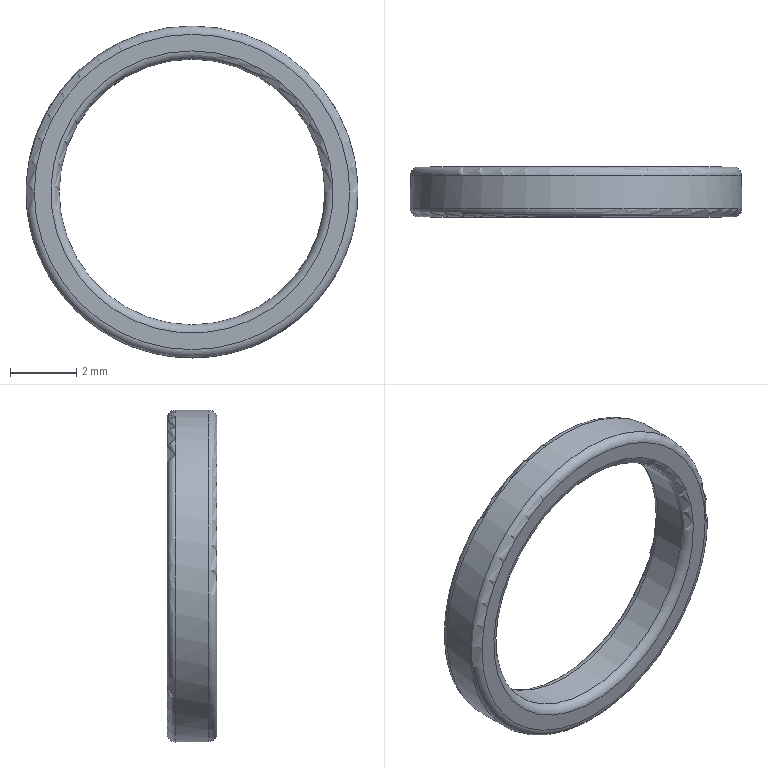Component | NX | AXLESPEEDWASHER | 1 solid | 8 faces | box 10 x 1.5 x 10 mm | volume 41 mm3 | torus 4 | plane 2 | cylinder 2 | commonest cylinder face diameters 10 x1 8 x1
STEP:
#1=CARTESIAN_POINT('',(0.,0.,0.));
#2=DIRECTION('',(0.,0.,1.));
#3=DIRECTION('',(1.,0.,0.));
#4=AXIS2_PLACEMENT_3D('',#1,#2,#3);
#5=CARTESIAN_POINT('',(-422.274,-112.,-59.25));
#6=VERTEX_POINT('',#5);
#7=CARTESIAN_POINT('',(-422.274,-112.,-63.5));
#8=DIRECTION('',(0.,1.,0.));
#9=DIRECTION('',(0.,0.,1.));
#10=AXIS2_PLACEMENT_3D('',#7,#8,#9);
#11=CIRCLE('',#10,4.25);
#12=CARTESIAN_POINT('',(-422.274,-112.,-63.5));
#13=DIRECTION('',(0.,-1.,0.));
#14=DIRECTION('',(0.,0.,1.));
#15=AXIS2_PLACEMENT_3D('',#12,#13,#14);
#16=PLANE('',#15);
#17=CARTESIAN_POINT('',(4.25,0.));
#18=CARTESIAN_POINT('',(4.25,-7.361));
#19=CARTESIAN_POINT('',(-2.125,-3.681));
#20=CARTESIAN_POINT('',(-8.5,-0.));
#21=CARTESIAN_POINT('',(-2.125,3.681));
#22=CARTESIAN_POINT('',(4.25,7.361));
#23=CARTESIAN_POINT('',(4.25,0.));
#24=(BOUNDED_CURVE()B_SPLINE_CURVE(2,(#17,#18,#19,#20,#21,#22,#23),.UNSPECIFIED.,.T.,.F.)B_SPLINE_CURVE_WITH_KNOTS((1,2,2,2,2,1),(-2.094,0.,2.094,4.189,6.283,8.378),.UNSPECIFIED.)CURVE()GEOMETRIC_REPRESENTATION_ITEM()RATIONAL_B_SPLINE_CURVE((1.,0.5,1.,0.5,1.,0.5,1.))REPRESENTATION_ITEM(''));
#25=(GEOMETRIC_REPRESENTATION_CONTEXT(2)PARAMETRIC_REPRESENTATION_CONTEXT()REPRESENTATION_CONTEXT('',''));
#26=DEFINITIONAL_REPRESENTATION('',(#24),#25);
#27=PCURVE('',#16,#26);
#28=CARTESIAN_POINT('',(-422.274,-111.75,-63.5));
#29=DIRECTION('',(0.,-1.,0.));
#30=DIRECTION('',(0.,0.,1.));
#31=AXIS2_PLACEMENT_3D('',#28,#29,#30);
#32=TOROIDAL_SURFACE('',#31,4.25,0.25);
#33=CARTESIAN_POINT('',(6.283,7.854));
#34=DIRECTION('',(-1.,0.));
#35=VECTOR('',#34,1.);
#36=LINE('',#33,#35);
#37=(GEOMETRIC_REPRESENTATION_CONTEXT(2)PARAMETRIC_REPRESENTATION_CONTEXT()REPRESENTATION_CONTEXT('',''));
#38=DEFINITIONAL_REPRESENTATION('',(#36),#37);
#39=PCURVE('',#32,#38);
#40=SURFACE_CURVE('',#11,(#27,#39),.PCURVE_S1.);
#41=EDGE_CURVE('',#6,#6,#40,.T.);
#42=ORIENTED_EDGE('',*,*,#41,.T.);
#43=EDGE_LOOP('',(#42));
#44=FACE_BOUND('',#43,.T.);
#45=CARTESIAN_POINT('',(-422.274,-112.,-58.75));
#46=VERTEX_POINT('',#45);
#47=CARTESIAN_POINT('',(-422.274,-112.,-63.5));
#48=DIRECTION('',(0.,-1.,0.));
#49=DIRECTION('',(0.,0.,1.));
#50=AXIS2_PLACEMENT_3D('',#47,#48,#49);
#51=CIRCLE('',#50,4.75);
#52=CARTESIAN_POINT('',(0.,0.));
#53=DIRECTION('',(1.,0.));
#54=AXIS2_PLACEMENT_2D('',#52,#53);
#55=CIRCLE('',#54,4.75);
#56=(GEOMETRIC_REPRESENTATION_CONTEXT(2)PARAMETRIC_REPRESENTATION_CONTEXT()REPRESENTATION_CONTEXT('',''));
#57=DEFINITIONAL_REPRESENTATION('',(#55),#56);
#58=PCURVE('',#16,#57);
#59=CARTESIAN_POINT('',(-422.274,-111.75,-63.5));
#60=DIRECTION('',(0.,-1.,0.));
#61=DIRECTION('',(0.,0.,1.));
#62=AXIS2_PLACEMENT_3D('',#59,#60,#61);
#63=TOROIDAL_SURFACE('',#62,4.75,0.25);
#64=CARTESIAN_POINT('',(0.,7.854));
#65=DIRECTION('',(1.,0.));
#66=VECTOR('',#65,1.);
#67=LINE('',#64,#66);
#68=(GEOMETRIC_REPRESENTATION_CONTEXT(2)PARAMETRIC_REPRESENTATION_CONTEXT()REPRESENTATION_CONTEXT('',''));
#69=DEFINITIONAL_REPRESENTATION('',(#67),#68);
#70=PCURVE('',#63,#69);
#71=SURFACE_CURVE('',#51,(#58,#70),.PCURVE_S1.);
#72=EDGE_CURVE('',#46,#46,#71,.T.);
#73=ORIENTED_EDGE('',*,*,#72,.T.);
#74=EDGE_LOOP('',(#73));
#75=FACE_BOUND('',#74,.T.);
#76=ADVANCED_FACE('',(#44,#75),#16,.T.);
#77=CARTESIAN_POINT('',(-422.274,-110.5,-67.75));
#78=VERTEX_POINT('',#77);
#79=CARTESIAN_POINT('',(-422.274,-110.5,-63.5));
#80=DIRECTION('',(0.,-1.,0.));
#81=DIRECTION('',(0.,0.,-1.));
#82=AXIS2_PLACEMENT_3D('',#79,#80,#81);
#83=CIRCLE('',#82,4.25);
#84=CARTESIAN_POINT('',(-422.274,-110.5,-63.5));
#85=DIRECTION('',(0.,1.,0.));
#86=DIRECTION('',(0.,0.,-1.));
#87=AXIS2_PLACEMENT_3D('',#84,#85,#86);
#88=PLANE('',#87);
#89=CARTESIAN_POINT('',(4.25,0.));
#90=CARTESIAN_POINT('',(4.25,-7.361));
#91=CARTESIAN_POINT('',(-2.125,-3.681));
#92=CARTESIAN_POINT('',(-8.5,-0.));
#93=CARTESIAN_POINT('',(-2.125,3.681));
#94=CARTESIAN_POINT('',(4.25,7.361));
#95=CARTESIAN_POINT('',(4.25,0.));
#96=(BOUNDED_CURVE()B_SPLINE_CURVE(2,(#89,#90,#91,#92,#93,#94,#95),.UNSPECIFIED.,.T.,.F.)B_SPLINE_CURVE_WITH_KNOTS((1,2,2,2,2,1),(-2.094,0.,2.094,4.189,6.283,8.378),.UNSPECIFIED.)CURVE()GEOMETRIC_REPRESENTATION_ITEM()RATIONAL_B_SPLINE_CURVE((1.,0.5,1.,0.5,1.,0.5,1.))REPRESENTATION_ITEM(''));
#97=(GEOMETRIC_REPRESENTATION_CONTEXT(2)PARAMETRIC_REPRESENTATION_CONTEXT()REPRESENTATION_CONTEXT('',''));
#98=DEFINITIONAL_REPRESENTATION('',(#96),#97);
#99=PCURVE('',#88,#98);
#100=CARTESIAN_POINT('',(-422.274,-110.75,-63.5));
#101=DIRECTION('',(0.,1.,0.));
#102=DIRECTION('',(0.,0.,-1.));
#103=AXIS2_PLACEMENT_3D('',#100,#101,#102);
#104=TOROIDAL_SURFACE('',#103,4.25,0.25);
#105=CARTESIAN_POINT('',(6.283,7.854));
#106=DIRECTION('',(-1.,0.));
#107=VECTOR('',#106,1.);
#108=LINE('',#105,#107);
#109=(GEOMETRIC_REPRESENTATION_CONTEXT(2)PARAMETRIC_REPRESENTATION_CONTEXT()REPRESENTATION_CONTEXT('',''));
#110=DEFINITIONAL_REPRESENTATION('',(#108),#109);
#111=PCURVE('',#104,#110);
#112=SURFACE_CURVE('',#83,(#99,#111),.PCURVE_S1.);
#113=EDGE_CURVE('',#78,#78,#112,.T.);
#114=ORIENTED_EDGE('',*,*,#113,.T.);
#115=EDGE_LOOP('',(#114));
#116=FACE_BOUND('',#115,.T.);
#117=CARTESIAN_POINT('',(-422.274,-110.5,-68.25));
#118=VERTEX_POINT('',#117);
#119=CARTESIAN_POINT('',(-422.274,-110.5,-63.5));
#120=DIRECTION('',(0.,1.,0.));
#121=DIRECTION('',(0.,0.,-1.));
#122=AXIS2_PLACEMENT_3D('',#119,#120,#121);
#123=CIRCLE('',#122,4.75);
#124=CARTESIAN_POINT('',(0.,0.));
#125=DIRECTION('',(1.,0.));
#126=AXIS2_PLACEMENT_2D('',#124,#125);
#127=CIRCLE('',#126,4.75);
#128=(GEOMETRIC_REPRESENTATION_CONTEXT(2)PARAMETRIC_REPRESENTATION_CONTEXT()REPRESENTATION_CONTEXT('',''));
#129=DEFINITIONAL_REPRESENTATION('',(#127),#128);
#130=PCURVE('',#88,#129);
#131=CARTESIAN_POINT('',(-422.274,-110.75,-63.5));
#132=DIRECTION('',(0.,1.,0.));
#133=DIRECTION('',(0.,0.,-1.));
#134=AXIS2_PLACEMENT_3D('',#131,#132,#133);
#135=TOROIDAL_SURFACE('',#134,4.75,0.25);
#136=CARTESIAN_POINT('',(0.,7.854));
#137=DIRECTION('',(1.,0.));
#138=VECTOR('',#137,1.);
#139=LINE('',#136,#138);
#140=(GEOMETRIC_REPRESENTATION_CONTEXT(2)PARAMETRIC_REPRESENTATION_CONTEXT()REPRESENTATION_CONTEXT('',''));
#141=DEFINITIONAL_REPRESENTATION('',(#139),#140);
#142=PCURVE('',#135,#141);
#143=SURFACE_CURVE('',#123,(#130,#142),.PCURVE_S1.);
#144=EDGE_CURVE('',#118,#118,#143,.T.);
#145=ORIENTED_EDGE('',*,*,#144,.T.);
#146=EDGE_LOOP('',(#145));
#147=FACE_BOUND('',#146,.T.);
#148=ADVANCED_FACE('',(#116,#147),#88,.T.);
#149=CARTESIAN_POINT('',(-422.274,-111.75,-58.5));
#150=VERTEX_POINT('',#149);
#151=CARTESIAN_POINT('',(-422.274,-111.75,-63.5));
#152=DIRECTION('',(0.,1.,0.));
#153=DIRECTION('',(0.,0.,1.));
#154=AXIS2_PLACEMENT_3D('',#151,#152,#153);
#155=CIRCLE('',#154,5.);
#156=CARTESIAN_POINT('',(-422.274,-110.5,-63.5));
#157=DIRECTION('',(0.,-1.,0.));
#158=DIRECTION('',(-1.,0.,0.));
#159=AXIS2_PLACEMENT_3D('',#156,#157,#158);
#160=CYLINDRICAL_SURFACE('',#159,5.);
#161=CARTESIAN_POINT('',(10.996,1.25));
#162=DIRECTION('',(-1.,0.));
#163=VECTOR('',#162,1.);
#164=LINE('',#161,#163);
#165=(GEOMETRIC_REPRESENTATION_CONTEXT(2)PARAMETRIC_REPRESENTATION_CONTEXT()REPRESENTATION_CONTEXT('',''));
#166=DEFINITIONAL_REPRESENTATION('',(#164),#165);
#167=PCURVE('',#160,#166);
#168=CARTESIAN_POINT('',(6.283,6.283));
#169=DIRECTION('',(-1.,0.));
#170=VECTOR('',#169,1.);
#171=LINE('',#168,#170);
#172=(GEOMETRIC_REPRESENTATION_CONTEXT(2)PARAMETRIC_REPRESENTATION_CONTEXT()REPRESENTATION_CONTEXT('',''));
#173=DEFINITIONAL_REPRESENTATION('',(#171),#172);
#174=PCURVE('',#63,#173);
#175=SURFACE_CURVE('',#155,(#167,#174),.PCURVE_S1.);
#176=EDGE_CURVE('',#150,#150,#175,.T.);
#177=ORIENTED_EDGE('',*,*,#176,.T.);
#178=CARTESIAN_POINT('',(-422.274,-110.75,-58.5));
#179=VERTEX_POINT('',#178);
#180=CARTESIAN_POINT('',(-422.274,-110.75,-58.5));
#181=CARTESIAN_POINT('',(-422.274,-111.75,-58.5));
#182=B_SPLINE_CURVE_WITH_KNOTS('',1,(#180,#181),.UNSPECIFIED.,.F.,.F.,(2,2),(0.25,1.25),.PIECEWISE_BEZIER_KNOTS.);
#183=CARTESIAN_POINT('',(4.712,0.));
#184=DIRECTION('',(0.,1.));
#185=VECTOR('',#184,1.);
#186=LINE('',#183,#185);
#187=(GEOMETRIC_REPRESENTATION_CONTEXT(2)PARAMETRIC_REPRESENTATION_CONTEXT()REPRESENTATION_CONTEXT('',''));
#188=DEFINITIONAL_REPRESENTATION('',(#186),#187);
#189=PCURVE('',#160,#188);
#190=CARTESIAN_POINT('',(10.996,0.));
#191=DIRECTION('',(0.,1.));
#192=VECTOR('',#191,1.);
#193=LINE('',#190,#192);
#194=(GEOMETRIC_REPRESENTATION_CONTEXT(2)PARAMETRIC_REPRESENTATION_CONTEXT()REPRESENTATION_CONTEXT('',''));
#195=DEFINITIONAL_REPRESENTATION('',(#193),#194);
#196=PCURVE('',#160,#195);
#197=SEAM_CURVE('',#182,(#189,#196),.PCURVE_S1.);
#198=EDGE_CURVE('',#179,#150,#197,.T.);
#199=ORIENTED_EDGE('',*,*,#198,.F.);
#200=CARTESIAN_POINT('',(-422.274,-110.75,-68.5));
#201=VERTEX_POINT('',#200);
#202=CARTESIAN_POINT('',(-422.274,-110.75,-63.5));
#203=DIRECTION('',(0.,-1.,0.));
#204=DIRECTION('',(0.,0.,-1.));
#205=AXIS2_PLACEMENT_3D('',#202,#203,#204);
#206=CIRCLE('',#205,5.);
#207=CARTESIAN_POINT('',(1.571,0.25));
#208=DIRECTION('',(1.,0.));
#209=VECTOR('',#208,1.);
#210=LINE('',#207,#209);
#211=(GEOMETRIC_REPRESENTATION_CONTEXT(2)PARAMETRIC_REPRESENTATION_CONTEXT()REPRESENTATION_CONTEXT('',''));
#212=DEFINITIONAL_REPRESENTATION('',(#210),#211);
#213=PCURVE('',#160,#212);
#214=CARTESIAN_POINT('',(6.283,6.283));
#215=DIRECTION('',(-1.,0.));
#216=VECTOR('',#215,1.);
#217=LINE('',#214,#216);
#218=(GEOMETRIC_REPRESENTATION_CONTEXT(2)PARAMETRIC_REPRESENTATION_CONTEXT()REPRESENTATION_CONTEXT('',''));
#219=DEFINITIONAL_REPRESENTATION('',(#217),#218);
#220=PCURVE('',#135,#219);
#221=SURFACE_CURVE('',#206,(#213,#220),.PCURVE_S1.);
#222=EDGE_CURVE('',#179,#201,#221,.T.);
#223=ORIENTED_EDGE('',*,*,#222,.T.);
#224=CARTESIAN_POINT('',(-422.274,-110.75,-63.5));
#225=DIRECTION('',(0.,-1.,0.));
#226=DIRECTION('',(0.,0.,-1.));
#227=AXIS2_PLACEMENT_3D('',#224,#225,#226);
#228=CIRCLE('',#227,5.);
#229=CARTESIAN_POINT('',(7.854,0.25));
#230=DIRECTION('',(1.,0.));
#231=VECTOR('',#230,1.);
#232=LINE('',#229,#231);
#233=(GEOMETRIC_REPRESENTATION_CONTEXT(2)PARAMETRIC_REPRESENTATION_CONTEXT()REPRESENTATION_CONTEXT('',''));
#234=DEFINITIONAL_REPRESENTATION('',(#232),#233);
#235=PCURVE('',#160,#234);
#236=CARTESIAN_POINT('',(6.283,6.283));
#237=DIRECTION('',(-1.,0.));
#238=VECTOR('',#237,1.);
#239=LINE('',#236,#238);
#240=(GEOMETRIC_REPRESENTATION_CONTEXT(2)PARAMETRIC_REPRESENTATION_CONTEXT()REPRESENTATION_CONTEXT('',''));
#241=DEFINITIONAL_REPRESENTATION('',(#239),#240);
#242=PCURVE('',#135,#241);
#243=SURFACE_CURVE('',#228,(#235,#242),.PCURVE_S1.);
#244=EDGE_CURVE('',#201,#179,#243,.T.);
#245=ORIENTED_EDGE('',*,*,#244,.T.);
#246=ORIENTED_EDGE('',*,*,#198,.T.);
#247=EDGE_LOOP('',(#177,#199,#223,#245,#246));
#248=FACE_BOUND('',#247,.T.);
#249=ADVANCED_FACE('',(#248),#160,.T.);
#250=CARTESIAN_POINT('',(-422.274,-110.75,-67.5));
#251=VERTEX_POINT('',#250);
#252=CARTESIAN_POINT('',(-422.274,-110.75,-63.5));
#253=DIRECTION('',(0.,1.,0.));
#254=DIRECTION('',(0.,0.,-1.));
#255=AXIS2_PLACEMENT_3D('',#252,#253,#254);
#256=CIRCLE('',#255,4.);
#257=CARTESIAN_POINT('',(-422.274,-112.,-63.5));
#258=DIRECTION('',(0.,1.,0.));
#259=DIRECTION('',(-1.,0.,0.));
#260=AXIS2_PLACEMENT_3D('',#257,#258,#259);
#261=CYLINDRICAL_SURFACE('',#260,4.);
#262=CARTESIAN_POINT('',(4.712,1.25));
#263=DIRECTION('',(1.,0.));
#264=VECTOR('',#263,1.);
#265=LINE('',#262,#264);
#266=(GEOMETRIC_REPRESENTATION_CONTEXT(2)PARAMETRIC_REPRESENTATION_CONTEXT()REPRESENTATION_CONTEXT('',''));
#267=DEFINITIONAL_REPRESENTATION('',(#265),#266);
#268=PCURVE('',#261,#267);
#269=CARTESIAN_POINT('',(0.,9.425));
#270=DIRECTION('',(1.,0.));
#271=VECTOR('',#270,1.);
#272=LINE('',#269,#271);
#273=(GEOMETRIC_REPRESENTATION_CONTEXT(2)PARAMETRIC_REPRESENTATION_CONTEXT()REPRESENTATION_CONTEXT('',''));
#274=DEFINITIONAL_REPRESENTATION('',(#272),#273);
#275=PCURVE('',#104,#274);
#276=SURFACE_CURVE('',#256,(#268,#275),.PCURVE_S1.);
#277=EDGE_CURVE('',#251,#251,#276,.T.);
#278=ORIENTED_EDGE('',*,*,#277,.F.);
#279=CARTESIAN_POINT('',(-422.274,-111.75,-67.5));
#280=VERTEX_POINT('',#279);
#281=CARTESIAN_POINT('',(-422.274,-111.75,-67.5));
#282=CARTESIAN_POINT('',(-422.274,-110.75,-67.5));
#283=B_SPLINE_CURVE_WITH_KNOTS('',1,(#281,#282),.UNSPECIFIED.,.F.,.F.,(2,2),(0.25,1.25),.PIECEWISE_BEZIER_KNOTS.);
#284=CARTESIAN_POINT('',(4.712,0.));
#285=DIRECTION('',(0.,1.));
#286=VECTOR('',#285,1.);
#287=LINE('',#284,#286);
#288=(GEOMETRIC_REPRESENTATION_CONTEXT(2)PARAMETRIC_REPRESENTATION_CONTEXT()REPRESENTATION_CONTEXT('',''));
#289=DEFINITIONAL_REPRESENTATION('',(#287),#288);
#290=PCURVE('',#261,#289);
#291=CARTESIAN_POINT('',(10.996,0.));
#292=DIRECTION('',(0.,1.));
#293=VECTOR('',#292,1.);
#294=LINE('',#291,#293);
#295=(GEOMETRIC_REPRESENTATION_CONTEXT(2)PARAMETRIC_REPRESENTATION_CONTEXT()REPRESENTATION_CONTEXT('',''));
#296=DEFINITIONAL_REPRESENTATION('',(#294),#295);
#297=PCURVE('',#261,#296);
#298=SEAM_CURVE('',#283,(#290,#297),.PCURVE_S1.);
#299=EDGE_CURVE('',#280,#251,#298,.T.);
#300=ORIENTED_EDGE('',*,*,#299,.F.);
#301=CARTESIAN_POINT('',(-422.274,-111.75,-59.5));
#302=VERTEX_POINT('',#301);
#303=CARTESIAN_POINT('',(-422.274,-111.75,-63.5));
#304=DIRECTION('',(0.,-1.,0.));
#305=DIRECTION('',(0.,0.,1.));
#306=AXIS2_PLACEMENT_3D('',#303,#304,#305);
#307=CIRCLE('',#306,4.);
#308=CARTESIAN_POINT('',(7.854,0.25));
#309=DIRECTION('',(-1.,0.));
#310=VECTOR('',#309,1.);
#311=LINE('',#308,#310);
#312=(GEOMETRIC_REPRESENTATION_CONTEXT(2)PARAMETRIC_REPRESENTATION_CONTEXT()REPRESENTATION_CONTEXT('',''));
#313=DEFINITIONAL_REPRESENTATION('',(#311),#312);
#314=PCURVE('',#261,#313);
#315=CARTESIAN_POINT('',(0.,9.425));
#316=DIRECTION('',(1.,-0.));
#317=VECTOR('',#316,1.);
#318=LINE('',#315,#317);
#319=(GEOMETRIC_REPRESENTATION_CONTEXT(2)PARAMETRIC_REPRESENTATION_CONTEXT()REPRESENTATION_CONTEXT('',''));
#320=DEFINITIONAL_REPRESENTATION('',(#318),#319);
#321=PCURVE('',#32,#320);
#322=SURFACE_CURVE('',#307,(#314,#321),.PCURVE_S1.);
#323=EDGE_CURVE('',#302,#280,#322,.T.);
#324=ORIENTED_EDGE('',*,*,#323,.F.);
#325=CARTESIAN_POINT('',(-422.274,-111.75,-63.5));
#326=DIRECTION('',(0.,-1.,0.));
#327=DIRECTION('',(0.,0.,1.));
#328=AXIS2_PLACEMENT_3D('',#325,#326,#327);
#329=CIRCLE('',#328,4.);
#330=CARTESIAN_POINT('',(14.137,0.25));
#331=DIRECTION('',(-1.,0.));
#332=VECTOR('',#331,1.);
#333=LINE('',#330,#332);
#334=(GEOMETRIC_REPRESENTATION_CONTEXT(2)PARAMETRIC_REPRESENTATION_CONTEXT()REPRESENTATION_CONTEXT('',''));
#335=DEFINITIONAL_REPRESENTATION('',(#333),#334);
#336=PCURVE('',#261,#335);
#337=CARTESIAN_POINT('',(0.,9.425));
#338=DIRECTION('',(1.,0.));
#339=VECTOR('',#338,1.);
#340=LINE('',#337,#339);
#341=(GEOMETRIC_REPRESENTATION_CONTEXT(2)PARAMETRIC_REPRESENTATION_CONTEXT()REPRESENTATION_CONTEXT('',''));
#342=DEFINITIONAL_REPRESENTATION('',(#340),#341);
#343=PCURVE('',#32,#342);
#344=SURFACE_CURVE('',#329,(#336,#343),.PCURVE_S1.);
#345=EDGE_CURVE('',#280,#302,#344,.T.);
#346=ORIENTED_EDGE('',*,*,#345,.F.);
#347=ORIENTED_EDGE('',*,*,#299,.T.);
#348=EDGE_LOOP('',(#278,#300,#324,#346,#347));
#349=FACE_BOUND('',#348,.F.);
#350=ADVANCED_FACE('',(#349),#261,.F.);
#351=ORIENTED_EDGE('',*,*,#277,.F.);
#352=CARTESIAN_POINT('',(-422.274,-110.5,-67.75));
#353=CARTESIAN_POINT('',(-422.274,-110.5,-67.683));
#354=CARTESIAN_POINT('',(-422.274,-110.521,-67.618));
#355=CARTESIAN_POINT('',(-422.274,-110.562,-67.562));
#356=CARTESIAN_POINT('',(-422.274,-110.618,-67.521));
#357=CARTESIAN_POINT('',(-422.274,-110.683,-67.5));
#358=CARTESIAN_POINT('',(-422.274,-110.75,-67.5));
#359=(BOUNDED_CURVE()B_SPLINE_CURVE(6,(#352,#353,#354,#355,#356,#357,#358),.UNSPECIFIED.,.F.,.F.)B_SPLINE_CURVE_WITH_KNOTS((7,7),(1.571,3.142),.PIECEWISE_BEZIER_KNOTS.)CURVE()GEOMETRIC_REPRESENTATION_ITEM()RATIONAL_B_SPLINE_CURVE((1.031,1.01,0.9979,0.994,0.9979,1.01,1.031))REPRESENTATION_ITEM(''));
#360=CARTESIAN_POINT('',(0.,6.283));
#361=DIRECTION('',(0.,1.));
#362=VECTOR('',#361,1.);
#363=LINE('',#360,#362);
#364=(GEOMETRIC_REPRESENTATION_CONTEXT(2)PARAMETRIC_REPRESENTATION_CONTEXT()REPRESENTATION_CONTEXT('',''));
#365=DEFINITIONAL_REPRESENTATION('',(#363),#364);
#366=PCURVE('',#104,#365);
#367=CARTESIAN_POINT('',(6.283,6.283));
#368=DIRECTION('',(0.,1.));
#369=VECTOR('',#368,1.);
#370=LINE('',#367,#369);
#371=(GEOMETRIC_REPRESENTATION_CONTEXT(2)PARAMETRIC_REPRESENTATION_CONTEXT()REPRESENTATION_CONTEXT('',''));
#372=DEFINITIONAL_REPRESENTATION('',(#370),#371);
#373=PCURVE('',#104,#372);
#374=SEAM_CURVE('',#359,(#366,#373),.PCURVE_S1.);
#375=EDGE_CURVE('',#78,#251,#374,.T.);
#376=ORIENTED_EDGE('',*,*,#375,.F.);
#377=ORIENTED_EDGE('',*,*,#113,.F.);
#378=ORIENTED_EDGE('',*,*,#375,.T.);
#379=EDGE_LOOP('',(#351,#376,#377,#378));
#380=FACE_BOUND('',#379,.T.);
#381=ADVANCED_FACE('',(#380),#104,.T.);
#382=ORIENTED_EDGE('',*,*,#323,.F.);
#383=CARTESIAN_POINT('',(-422.274,-112.,-59.25));
#384=CARTESIAN_POINT('',(-422.274,-112.,-59.317));
#385=CARTESIAN_POINT('',(-422.274,-111.979,-59.382));
#386=CARTESIAN_POINT('',(-422.274,-111.938,-59.438));
#387=CARTESIAN_POINT('',(-422.274,-111.882,-59.479));
#388=CARTESIAN_POINT('',(-422.274,-111.817,-59.5));
#389=CARTESIAN_POINT('',(-422.274,-111.75,-59.5));
#390=(BOUNDED_CURVE()B_SPLINE_CURVE(6,(#383,#384,#385,#386,#387,#388,#389),.UNSPECIFIED.,.F.,.F.)B_SPLINE_CURVE_WITH_KNOTS((7,7),(1.571,3.142),.PIECEWISE_BEZIER_KNOTS.)CURVE()GEOMETRIC_REPRESENTATION_ITEM()RATIONAL_B_SPLINE_CURVE((1.031,1.01,0.9979,0.994,0.9979,1.01,1.031))REPRESENTATION_ITEM(''));
#391=CARTESIAN_POINT('',(0.,6.283));
#392=DIRECTION('',(0.,1.));
#393=VECTOR('',#392,1.);
#394=LINE('',#391,#393);
#395=(GEOMETRIC_REPRESENTATION_CONTEXT(2)PARAMETRIC_REPRESENTATION_CONTEXT()REPRESENTATION_CONTEXT('',''));
#396=DEFINITIONAL_REPRESENTATION('',(#394),#395);
#397=PCURVE('',#32,#396);
#398=CARTESIAN_POINT('',(6.283,6.283));
#399=DIRECTION('',(0.,1.));
#400=VECTOR('',#399,1.);
#401=LINE('',#398,#400);
#402=(GEOMETRIC_REPRESENTATION_CONTEXT(2)PARAMETRIC_REPRESENTATION_CONTEXT()REPRESENTATION_CONTEXT('',''));
#403=DEFINITIONAL_REPRESENTATION('',(#401),#402);
#404=PCURVE('',#32,#403);
#405=SEAM_CURVE('',#390,(#397,#404),.PCURVE_S1.);
#406=EDGE_CURVE('',#6,#302,#405,.T.);
#407=ORIENTED_EDGE('',*,*,#406,.F.);
#408=ORIENTED_EDGE('',*,*,#41,.F.);
#409=ORIENTED_EDGE('',*,*,#406,.T.);
#410=ORIENTED_EDGE('',*,*,#345,.F.);
#411=EDGE_LOOP('',(#382,#407,#408,#409,#410));
#412=FACE_BOUND('',#411,.T.);
#413=ADVANCED_FACE('',(#412),#32,.T.);
#414=ORIENTED_EDGE('',*,*,#72,.F.);
#415=CARTESIAN_POINT('',(-422.274,-111.75,-58.5));
#416=CARTESIAN_POINT('',(-422.274,-111.817,-58.5));
#417=CARTESIAN_POINT('',(-422.274,-111.882,-58.521));
#418=CARTESIAN_POINT('',(-422.274,-111.938,-58.562));
#419=CARTESIAN_POINT('',(-422.274,-111.979,-58.618));
#420=CARTESIAN_POINT('',(-422.274,-112.,-58.683));
#421=CARTESIAN_POINT('',(-422.274,-112.,-58.75));
#422=(BOUNDED_CURVE()B_SPLINE_CURVE(6,(#415,#416,#417,#418,#419,#420,#421),.UNSPECIFIED.,.F.,.F.)B_SPLINE_CURVE_WITH_KNOTS((7,7),(0.,1.571),.PIECEWISE_BEZIER_KNOTS.)CURVE()GEOMETRIC_REPRESENTATION_ITEM()RATIONAL_B_SPLINE_CURVE((1.031,1.01,0.9979,0.994,0.9979,1.01,1.031))REPRESENTATION_ITEM(''));
#423=CARTESIAN_POINT('',(0.,6.283));
#424=DIRECTION('',(0.,1.));
#425=VECTOR('',#424,1.);
#426=LINE('',#423,#425);
#427=(GEOMETRIC_REPRESENTATION_CONTEXT(2)PARAMETRIC_REPRESENTATION_CONTEXT()REPRESENTATION_CONTEXT('',''));
#428=DEFINITIONAL_REPRESENTATION('',(#426),#427);
#429=PCURVE('',#63,#428);
#430=CARTESIAN_POINT('',(6.283,6.283));
#431=DIRECTION('',(0.,1.));
#432=VECTOR('',#431,1.);
#433=LINE('',#430,#432);
#434=(GEOMETRIC_REPRESENTATION_CONTEXT(2)PARAMETRIC_REPRESENTATION_CONTEXT()REPRESENTATION_CONTEXT('',''));
#435=DEFINITIONAL_REPRESENTATION('',(#433),#434);
#436=PCURVE('',#63,#435);
#437=SEAM_CURVE('',#422,(#429,#436),.PCURVE_S1.);
#438=EDGE_CURVE('',#150,#46,#437,.T.);
#439=ORIENTED_EDGE('',*,*,#438,.F.);
#440=ORIENTED_EDGE('',*,*,#176,.F.);
#441=ORIENTED_EDGE('',*,*,#438,.T.);
#442=EDGE_LOOP('',(#414,#439,#440,#441));
#443=FACE_BOUND('',#442,.T.);
#444=ADVANCED_FACE('',(#443),#63,.T.);
#445=ORIENTED_EDGE('',*,*,#144,.F.);
#446=CARTESIAN_POINT('',(-422.274,-110.75,-68.5));
#447=CARTESIAN_POINT('',(-422.274,-110.683,-68.5));
#448=CARTESIAN_POINT('',(-422.274,-110.618,-68.479));
#449=CARTESIAN_POINT('',(-422.274,-110.562,-68.438));
#450=CARTESIAN_POINT('',(-422.274,-110.521,-68.382));
#451=CARTESIAN_POINT('',(-422.274,-110.5,-68.317));
#452=CARTESIAN_POINT('',(-422.274,-110.5,-68.25));
#453=(BOUNDED_CURVE()B_SPLINE_CURVE(6,(#446,#447,#448,#449,#450,#451,#452),.UNSPECIFIED.,.F.,.F.)B_SPLINE_CURVE_WITH_KNOTS((7,7),(0.,1.571),.PIECEWISE_BEZIER_KNOTS.)CURVE()GEOMETRIC_REPRESENTATION_ITEM()RATIONAL_B_SPLINE_CURVE((1.031,1.01,0.9979,0.994,0.9979,1.01,1.031))REPRESENTATION_ITEM(''));
#454=CARTESIAN_POINT('',(0.,6.283));
#455=DIRECTION('',(0.,1.));
#456=VECTOR('',#455,1.);
#457=LINE('',#454,#456);
#458=(GEOMETRIC_REPRESENTATION_CONTEXT(2)PARAMETRIC_REPRESENTATION_CONTEXT()REPRESENTATION_CONTEXT('',''));
#459=DEFINITIONAL_REPRESENTATION('',(#457),#458);
#460=PCURVE('',#135,#459);
#461=CARTESIAN_POINT('',(6.283,6.283));
#462=DIRECTION('',(0.,1.));
#463=VECTOR('',#462,1.);
#464=LINE('',#461,#463);
#465=(GEOMETRIC_REPRESENTATION_CONTEXT(2)PARAMETRIC_REPRESENTATION_CONTEXT()REPRESENTATION_CONTEXT('',''));
#466=DEFINITIONAL_REPRESENTATION('',(#464),#465);
#467=PCURVE('',#135,#466);
#468=SEAM_CURVE('',#453,(#460,#467),.PCURVE_S1.);
#469=EDGE_CURVE('',#201,#118,#468,.T.);
#470=ORIENTED_EDGE('',*,*,#469,.F.);
#471=ORIENTED_EDGE('',*,*,#222,.F.);
#472=ORIENTED_EDGE('',*,*,#244,.F.);
#473=ORIENTED_EDGE('',*,*,#469,.T.);
#474=EDGE_LOOP('',(#445,#470,#471,#472,#473));
#475=FACE_BOUND('',#474,.T.);
#476=ADVANCED_FACE('',(#475),#135,.T.);
#477=CLOSED_SHELL('',(#76,#148,#249,#350,#381,#413,#444,#476));
#478=MANIFOLD_SOLID_BREP('',#477);
#479=(LENGTH_UNIT()NAMED_UNIT(*)SI_UNIT(.MILLI.,.METRE.));
#480=UNCERTAINTY_MEASURE_WITH_UNIT(LENGTH_MEASURE(0.00001),#479,'','');
#481=(NAMED_UNIT(*)PLANE_ANGLE_UNIT()SI_UNIT($,.RADIAN.));
#482=(NAMED_UNIT(*)SI_UNIT($,.STERADIAN.)SOLID_ANGLE_UNIT());
#483=(GEOMETRIC_REPRESENTATION_CONTEXT(3)GLOBAL_UNCERTAINTY_ASSIGNED_CONTEXT((#480))GLOBAL_UNIT_ASSIGNED_CONTEXT((#479,#481,#482))REPRESENTATION_CONTEXT('',''));
#484=ADVANCED_BREP_SHAPE_REPRESENTATION('',(#4,#478),#483);